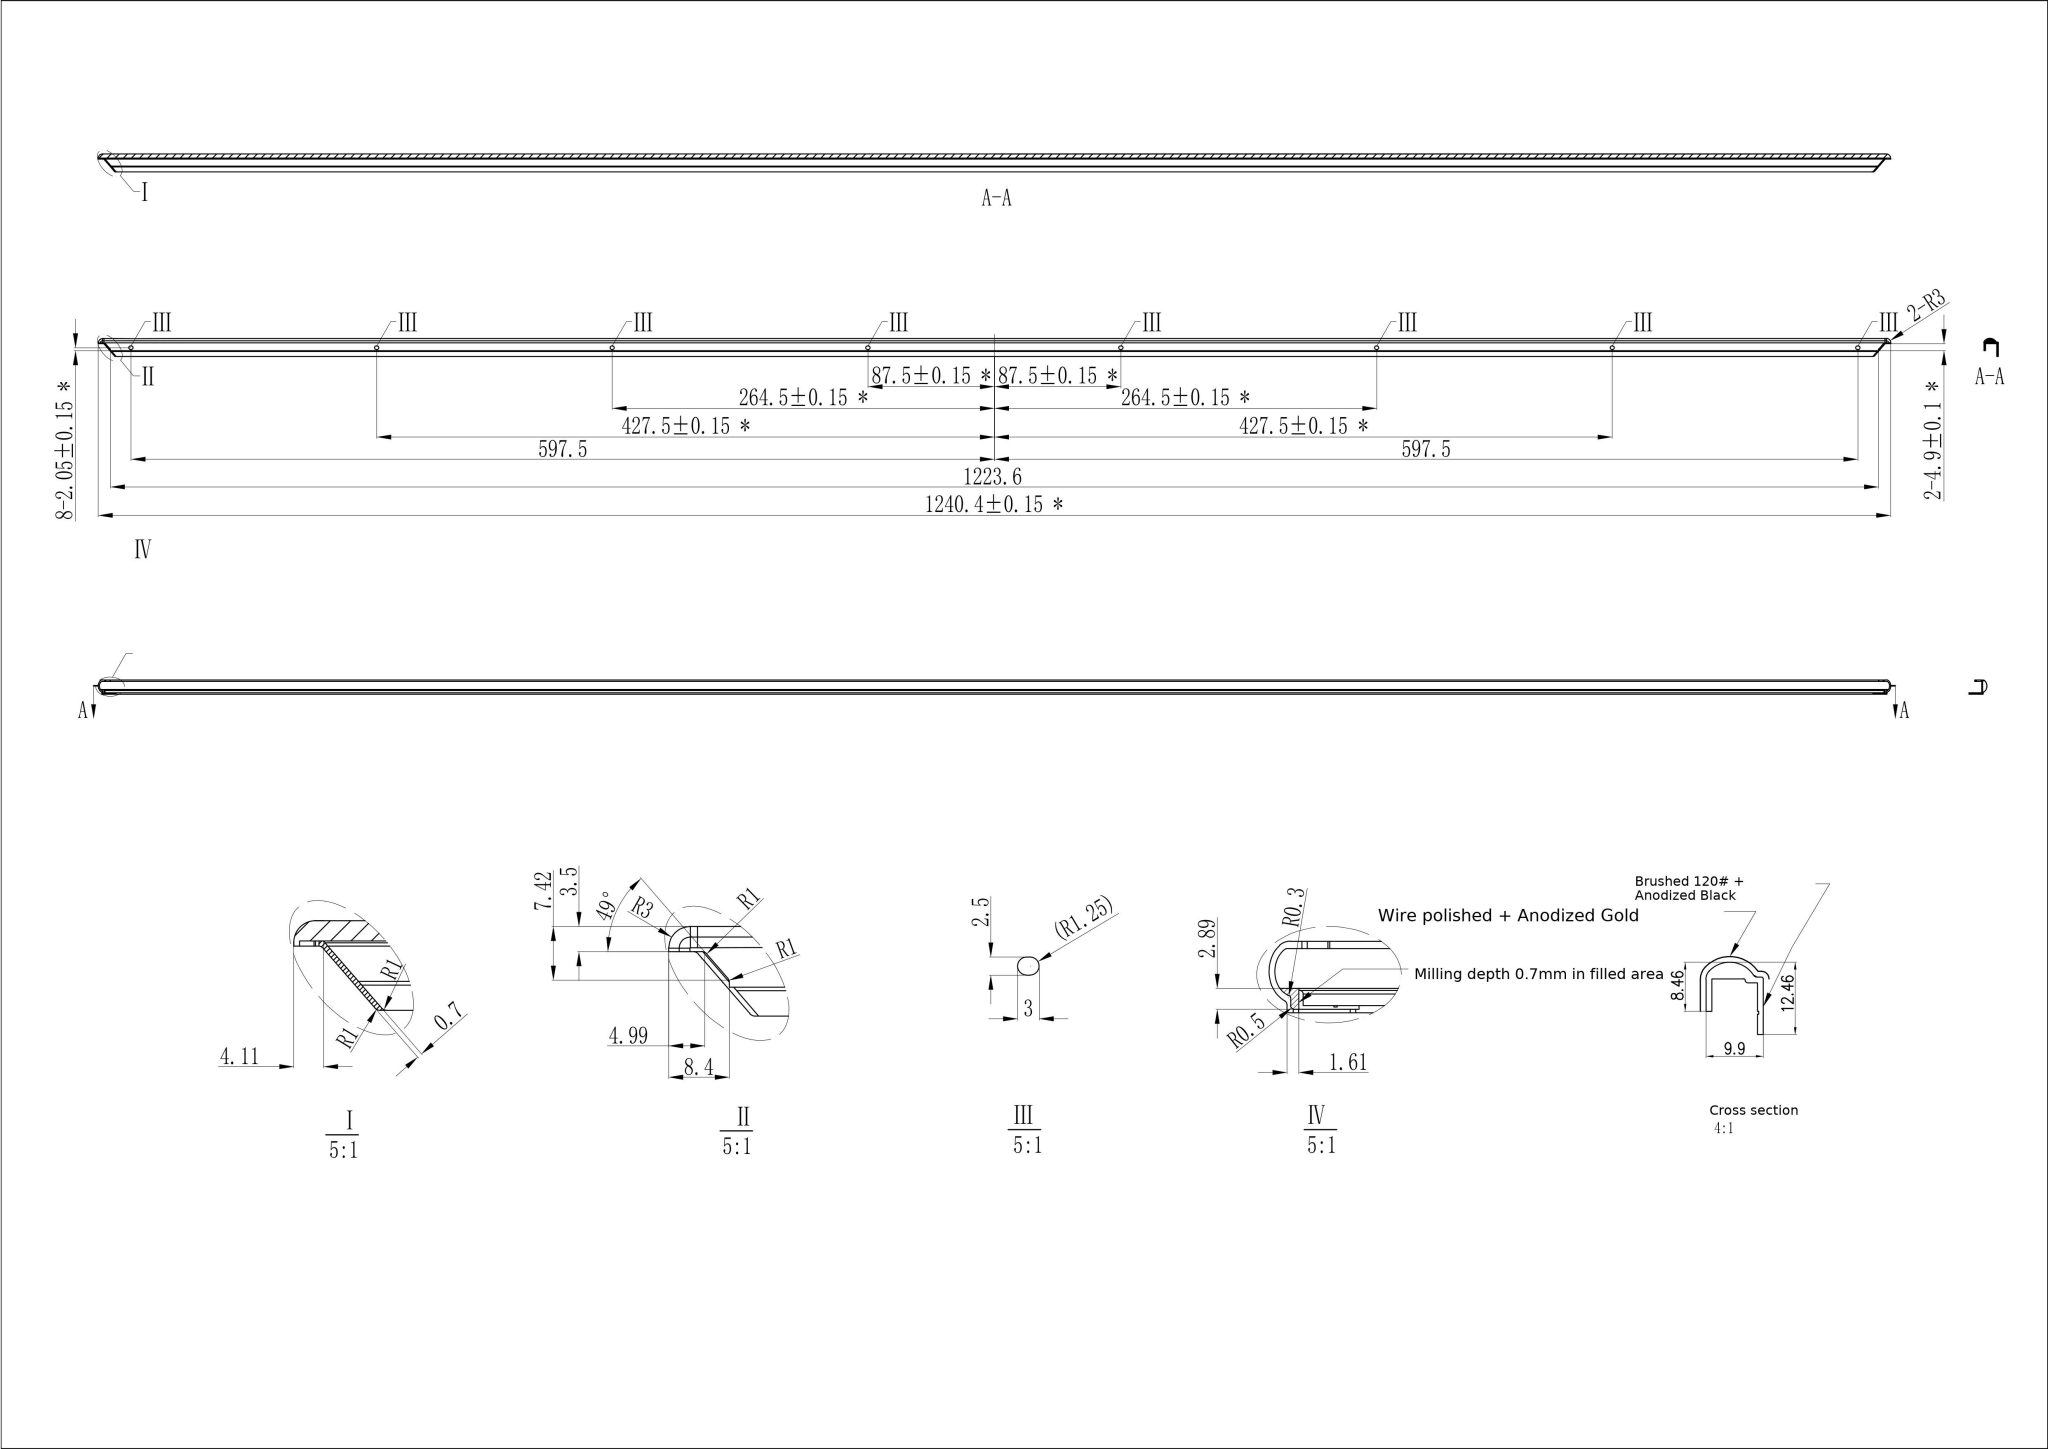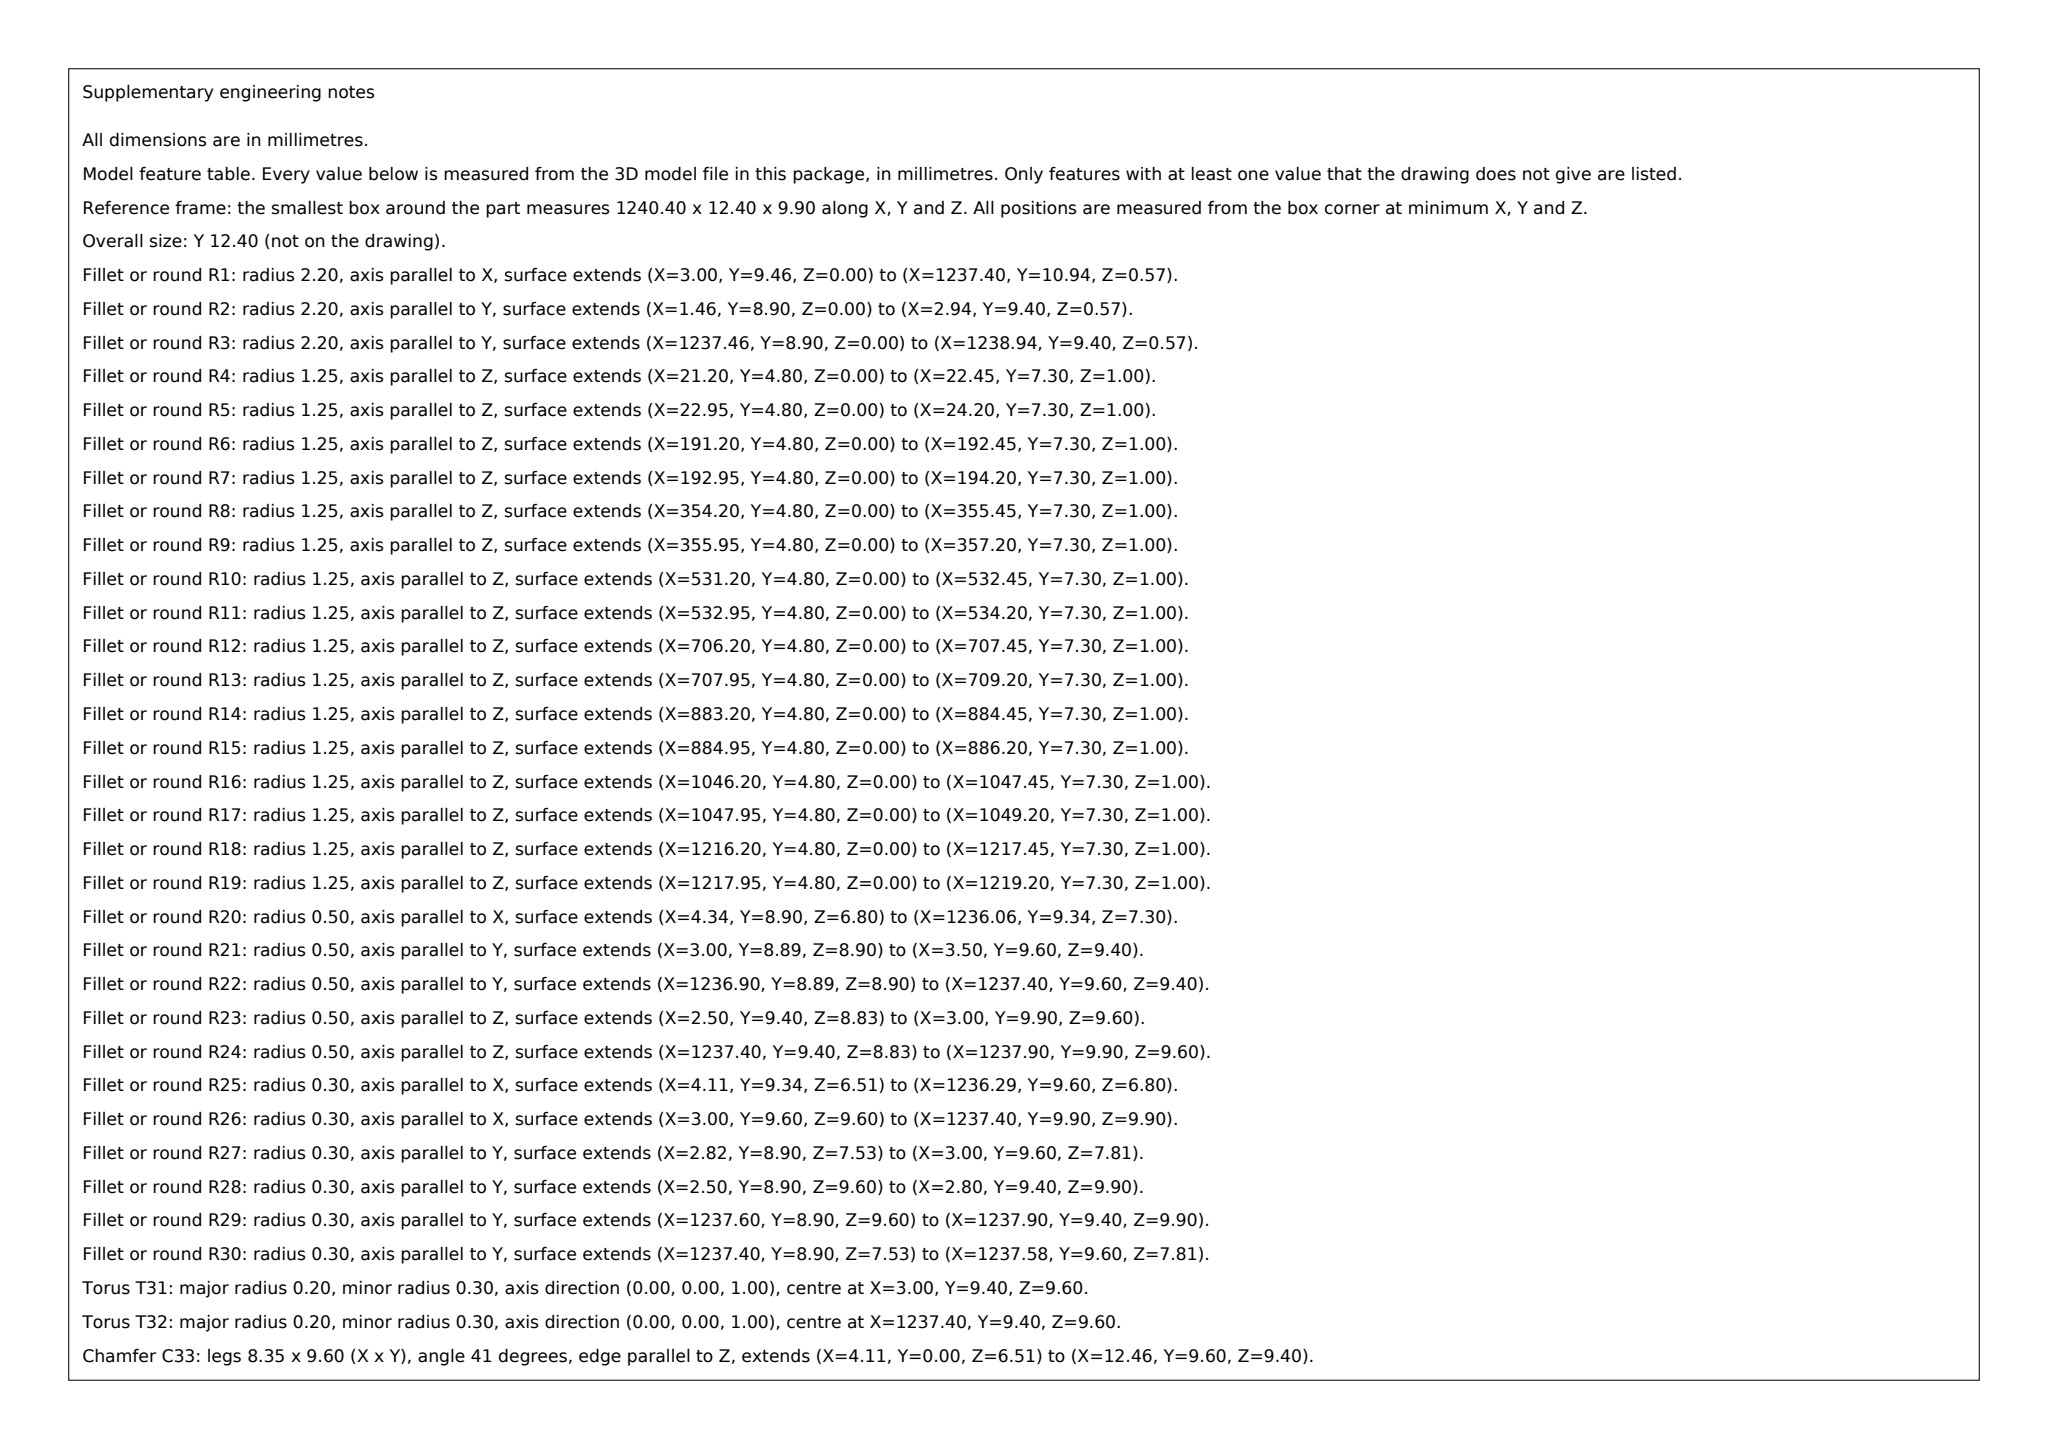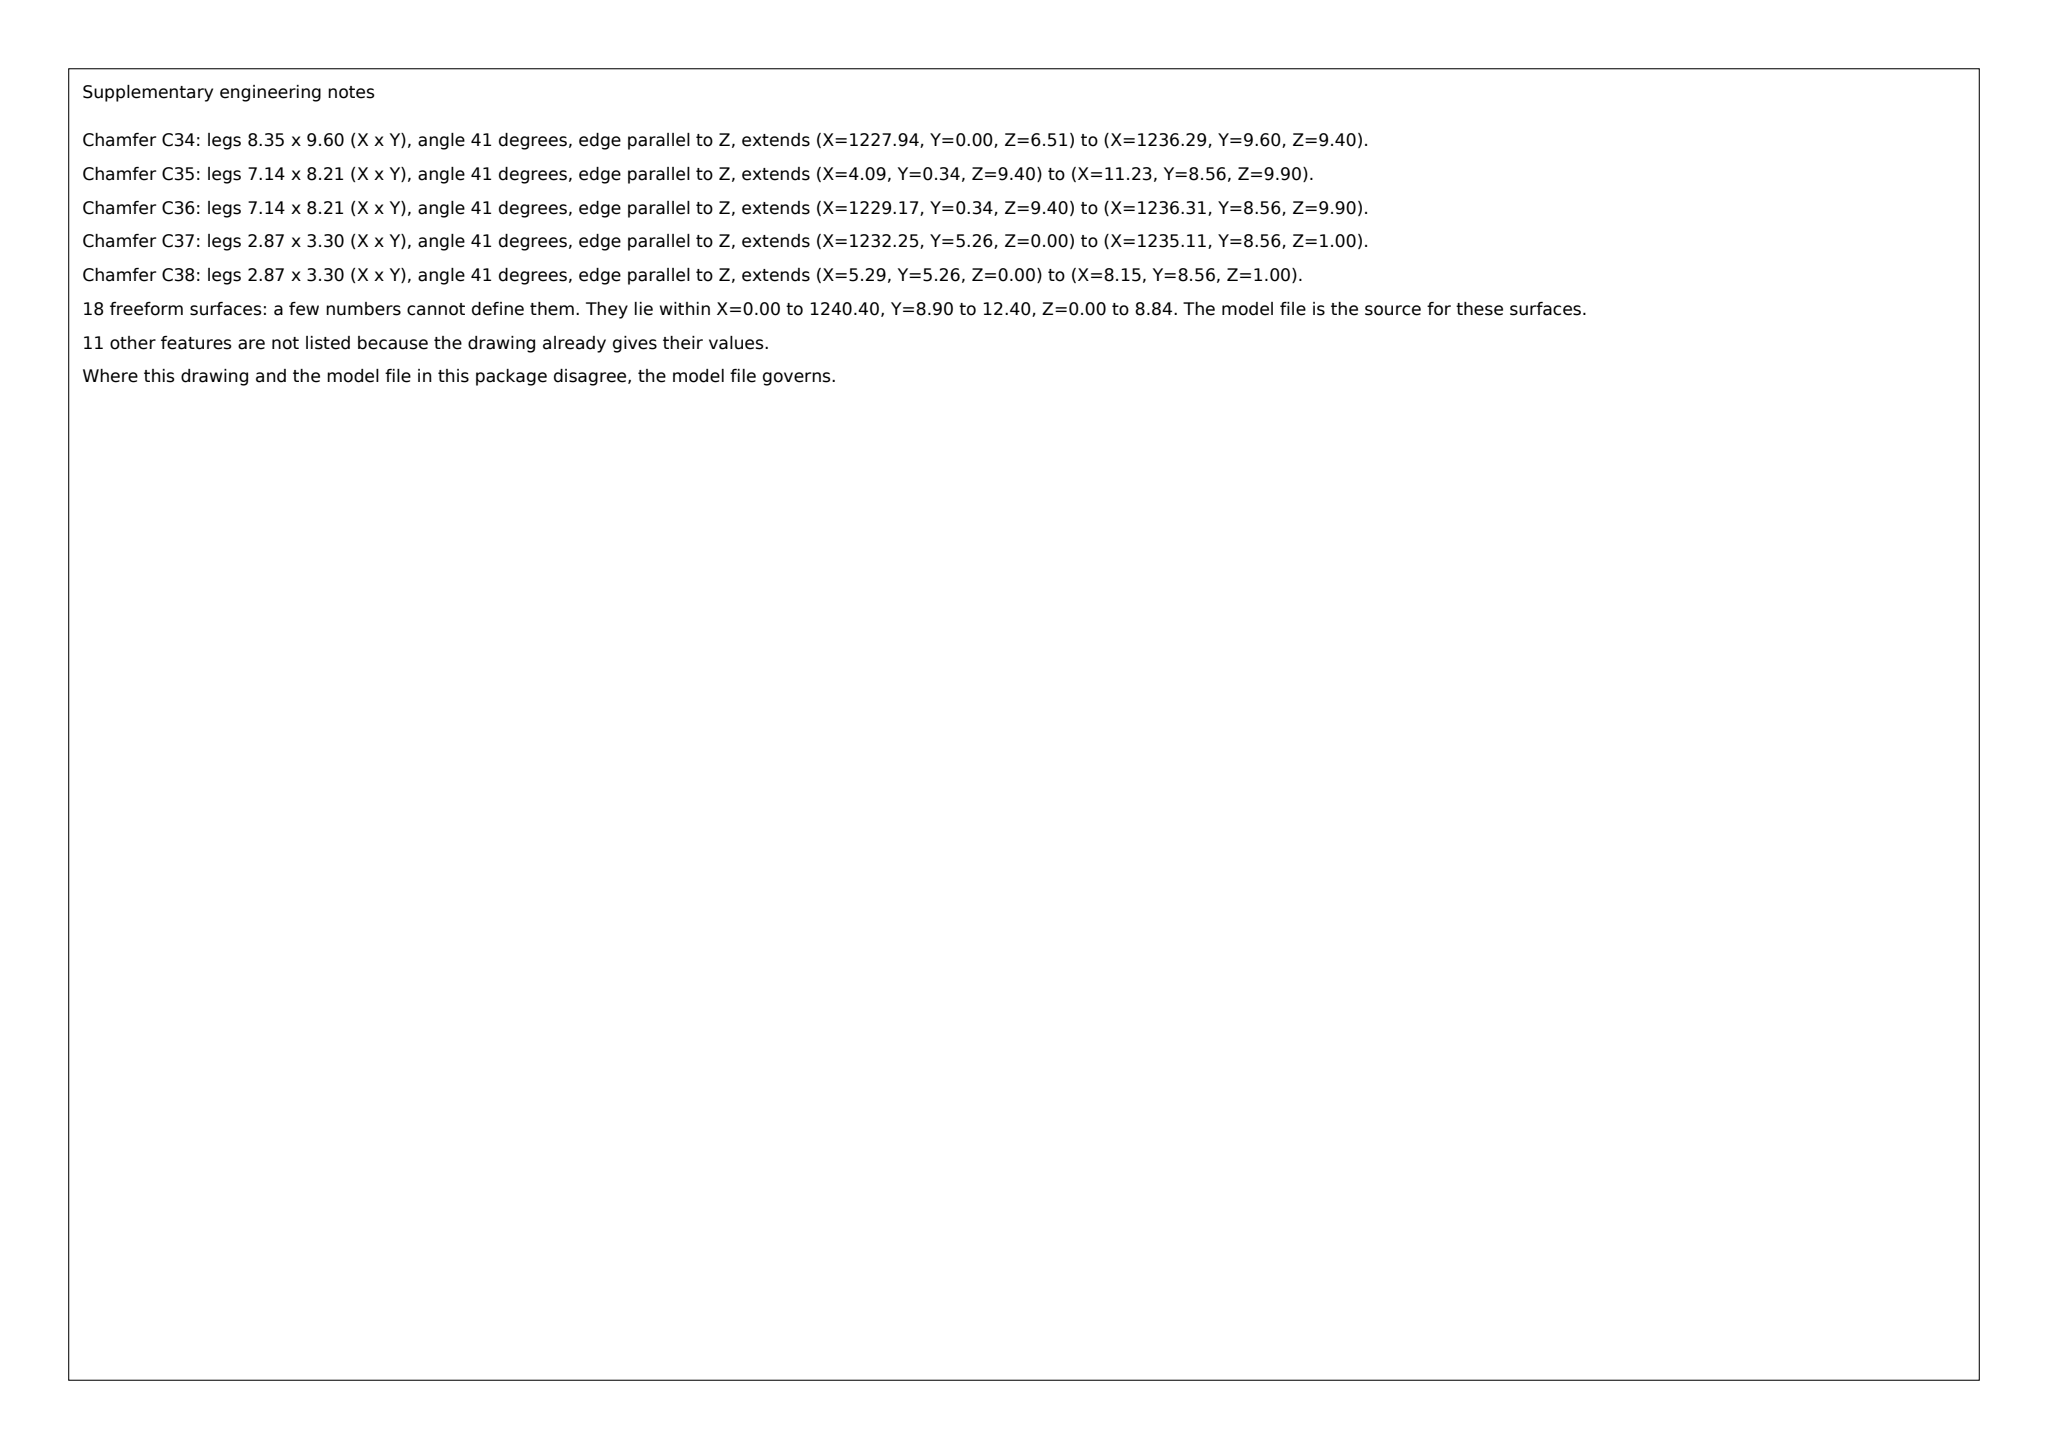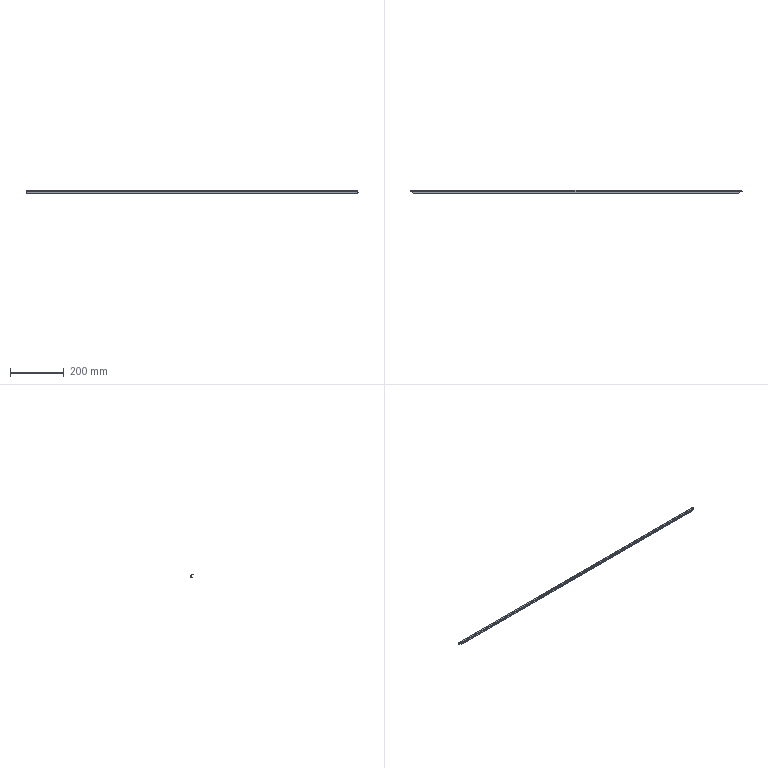Part | SolidWorks | mm | 1 solid | 116 faces | box 1240.4 x 12.4 x 9.9 mm | volume 43095 mm3 | cylinder 51 | plane 45 | spline 18 | torus 2 | commonest cylinder face diameters 2.5 x24 2 x8 0.6 x6 1 x5 1.4 x4 4.4 x4